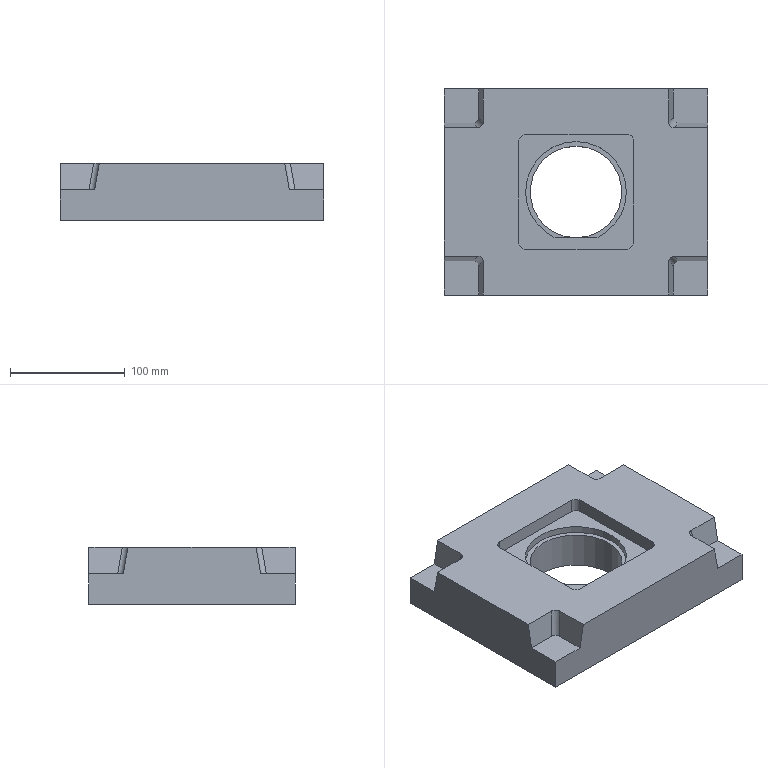CAM job | NX | mm | 3-axis | 1 set-up | 2 operations | part box 230 x 180 x 50
set-up 1
1. Cavity Milling | Mill Mill5 D16 | CAVITY_MILL | path 10991.743 mm | 27.099 min
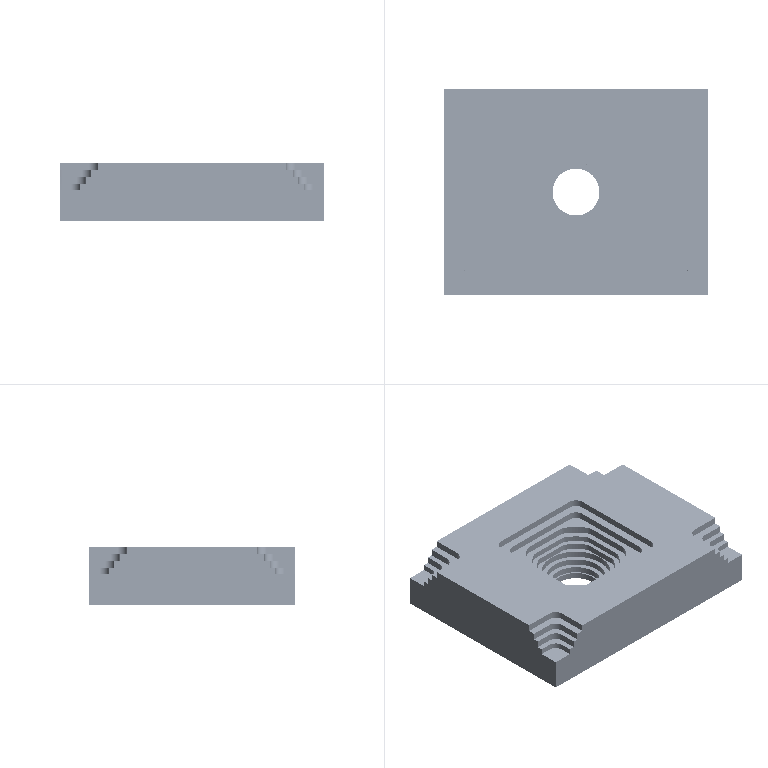2. Cavity Milling | Mill Mill5 D16 | CAVITY_MILL_COPY | path 10991.743 mm | 27.099 min